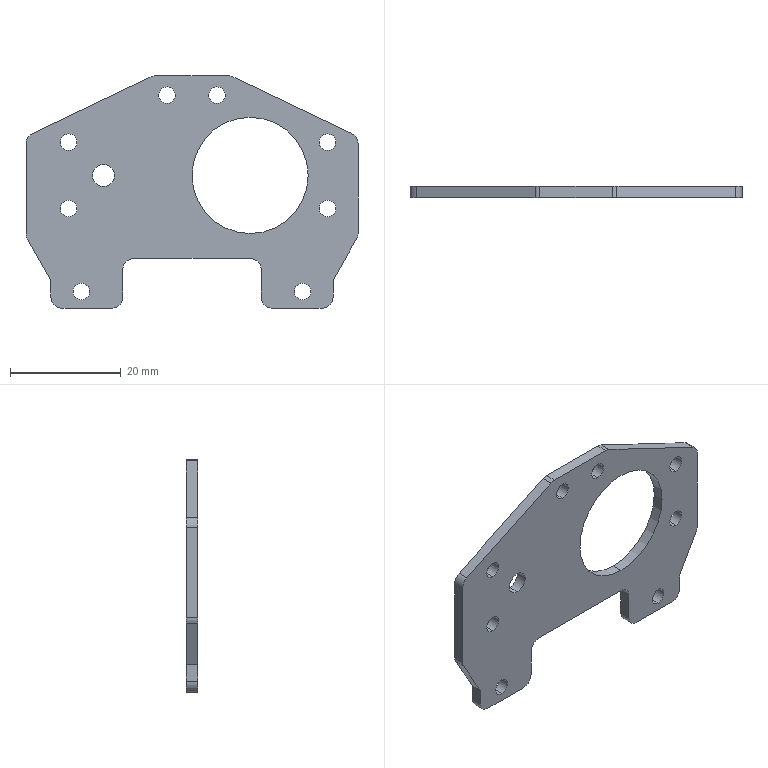Component | SolidWorks | 4-2 | 1 solid | 48 faces | box 60 x 2 x 42 mm | volume 3088 mm3 | cylinder 32 | plane 16 | commonest cylinder face diameters 3 x16 4 x14 21 x2
build123d program:
from build123d import *

# Parameters (mm, degrees)
SKETCH1_W           = 60
SKETCH1_H           = 42
BOSS_EXTRUDE1_DEPTH = 2
SKETCH2_W           = 25
SKETCH2_H           = 9
CUT_EXTRUDE1_DEPTH  = 2
CUT_EXTRUDE2_DEPTH  = 2
CUT_EXTRUDE3_DEPTH  = 2
SKETCH5_R           = 2
SKETCH5_R_2         = 10.5
SKETCH5_R_3         = 1.5
CUT_EXTRUDE4_DEPTH  = 10
FILLET1_R           = 2
SKETCH6_R           = 1.5
CUT_EXTRUDE5_DEPTH  = 10


with BuildPart() as part:
    # Sketch1 → Boss-Extrude1 (new body)
    with BuildSketch(Plane(origin=(0, 0, 0), x_dir=(1, 0, 0), z_dir=(0, 1, 0))):
        Rectangle(SKETCH1_W, SKETCH1_H)
    extrude(amount=BOSS_EXTRUDE1_DEPTH)

    # Sketch2 → Cut-Extrude1 (cut)
    with BuildSketch(Plane(origin=(0, 2, 0), x_dir=(1, 0, 0), z_dir=(0, 1, 0))):
        with Locations((0, 16.5)):
            Rectangle(SKETCH2_W, SKETCH2_H)
    extrude(amount=-CUT_EXTRUDE1_DEPTH, mode=Mode.SUBTRACT)

    # Sketch3 → Cut-Extrude2 (cut)
    with BuildSketch(Plane(origin=(0, 2, 0), x_dir=(1, 0, 0), z_dir=(0, 1, 0))):
        Polygon((25.5, 21), (25.5, 16), (30, 8), (30, 21), align=None)
        Polygon((-25.5, 21), (-25.5, 16), (-30.037, 8), (-30, 21), align=None)
    extrude(amount=-CUT_EXTRUDE2_DEPTH, mode=Mode.SUBTRACT)

    # Sketch4 → Cut-Extrude3 (cut)
    with BuildSketch(Plane(origin=(0, 2, 0), x_dir=(1, 0, 0), z_dir=(0, 1, 0))):
        Polygon((30.075, -10), (7, -21), (30, -21), align=None)
        Polygon((-30.045, -10), (-7, -21), (-30, -21), align=None)
    extrude(amount=-CUT_EXTRUDE3_DEPTH, mode=Mode.SUBTRACT)

    # Sketch5 → Cut-Extrude4 (cut)
    with BuildSketch(Plane(origin=(0, 2, 0), x_dir=(1, 0, 0), z_dir=(0, 1, 0))):
        with Locations(Location((-16, -3, 0), (0, 0, 270))):
            Circle(SKETCH5_R)
        with Locations(Location((10.5, -3, 0), (0, 0, 270))):
            Circle(SKETCH5_R_2)
        with Locations(Location((-22.28, 3, 0), (0, 0, 270))):
            Circle(SKETCH5_R_3)
        with Locations(Location((-22.28, -9, 0), (0, 0, 270))):
            Circle(SKETCH5_R_3)
        with Locations(Location((24.5, 3, 0), (0, 0, 270))):
            Circle(SKETCH5_R_3)
        with Locations(Location((24.5, -9, 0), (0, 0, 270))):
            Circle(SKETCH5_R_3)
        with Locations(Location((-4.5, -17.5, 0), (0, 0, 270))):
            Circle(SKETCH5_R_3)
        with Locations(Location((4.5, -17.5, 0), (0, 0, 270))):
            Circle(SKETCH5_R_3)
    extrude(amount=-CUT_EXTRUDE4_DEPTH, mode=Mode.SUBTRACT)

    # Fillet1
    fillet1_edges = [part.edges().sort_by_distance(p)[0] for p in [
        (-12.5, 1, -21),
        (12.5, 1, -21),
        (12.5, 1, -12),
        (-12.5, 1, -12),
        (25.5, 1, -21),
        (30, 1, -8),
        (-30, 1, -8.065),
        (-25.5, 1, -21),
        (30, 1, 10.036),
        (7, 1, 21),
        (-30, 1, 10.022),
        (-7, 1, 21),
    ]]
    fillet(fillet1_edges, radius=FILLET1_R)

    # Sketch6 → Cut-Extrude5 (cut)
    with BuildSketch(Plane(origin=(0, 2, 0), x_dir=(1, 0, 0), z_dir=(0, 1, 0))):
        with Locations(Location((20, 18, 0), (0, 0, 270))):
            Circle(SKETCH6_R)
        with Locations(Location((-20, 18, 0), (0, 0, 270))):
            Circle(SKETCH6_R)
    extrude(amount=-CUT_EXTRUDE5_DEPTH, mode=Mode.SUBTRACT)


solid = part.part

# Placed as in the assembly
solid = solid.moved(Location((-1.765, 16.631, 51), (0, 0, 0)))